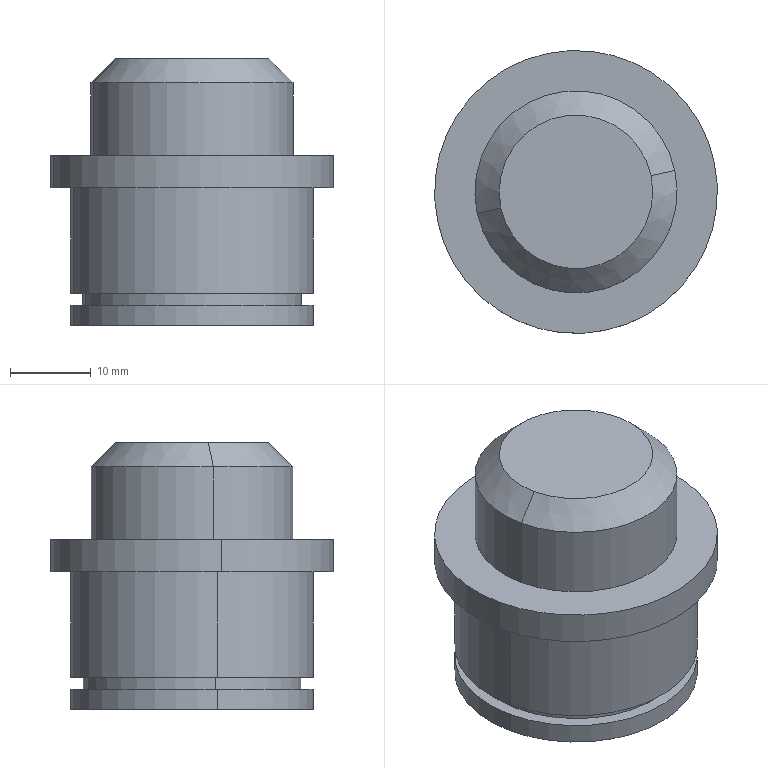Component | SolidWorks | 12AOuterSideWheel-EngravingAndMillingAxis-1_12AOuterSideWheelSmallAxis-1 | 1 solid | 18 faces | box 35 x 35 x 33 mm | volume 21229 mm3 | cylinder 10 | plane 6 | cone 2 | commonest cylinder face diameters 30 x4 27 x2 35 x2 25 x2 | material Cr12MoV
build123d program:
from build123d import *

# Parameters (mm, degrees)
SKETCH1_R           = 12.5
BOSS_EXTRUDE1_DEPTH = 12
SKETCH2_R           = 17.5
BOSS_EXTRUDE2_DEPTH = 4
SKETCH3_R           = 15
BOSS_EXTRUDE3_DEPTH = 17
SKETCH4_W           = 1.5
SKETCH4_H           = 1.5
CHAMFER1_SIZE       = 3


with BuildPart() as part:
    # Sketch1 → Boss-Extrude1 (new body)
    with BuildSketch(Plane.XY):
        Circle(SKETCH1_R)
    extrude(amount=BOSS_EXTRUDE1_DEPTH)

    # Sketch2 → Boss-Extrude2 (add)
    with BuildSketch(Plane.XY.offset(12)):
        Circle(SKETCH2_R)
    extrude(amount=BOSS_EXTRUDE2_DEPTH)

    # Sketch3 → Boss-Extrude3 (add)
    with BuildSketch(Plane.XY.offset(16)):
        Circle(SKETCH3_R)
    extrude(amount=BOSS_EXTRUDE3_DEPTH)

    # Sketch4 → Cut-Revolve1 (revolve, cut)
    with BuildSketch(Plane(origin=(0, 0, 0), x_dir=(1, 0, 0), z_dir=(0, 1, 0))):
        with Locations((14.25, -29.75)):
            Rectangle(SKETCH4_W, SKETCH4_H)
    revolve(axis=Axis((0, 0, 33), (0, 0, -1)), mode=Mode.SUBTRACT)

    # Chamfer1
    chamfer1_edges = [part.edges().sort_by_distance(p)[0] for p in [
        (-12.5, 0, 0),
    ]]
    chamfer(chamfer1_edges, length=CHAMFER1_SIZE)


solid = part.part

# Placed as in the assembly
solid = solid.moved(Location((271.598, 136.538, 72.25), (180, 0, 0)))
STEP:
#1=CARTESIAN_POINT('',(11.058,5.455,2.844));
#2=VERTEX_POINT('',#1);
#3=CARTESIAN_POINT('',(10.327,5.296,2.844));
#4=VERTEX_POINT('',#3);
#5=CARTESIAN_POINT('',(10.693,5.376,2.844));
#6=DIRECTION('',(0.,0.,1.));
#7=DIRECTION('',(-0.9774,-0.2113,0.));
#8=AXIS2_PLACEMENT_3D('',#5,#6,#7);
#9=CIRCLE('',#8,0.374);
#10=EDGE_CURVE('',#2,#4,#9,.T.);
#11=ORIENTED_EDGE('',*,*,#10,.F.);
#12=CARTESIAN_POINT('',(11.174,5.48,2.726));
#13=VERTEX_POINT('',#12);
#14=CARTESIAN_POINT('',(11.174,5.48,2.726));
#15=DIRECTION('',(0.6911,0.1494,-0.7071));
#16=VECTOR('',#15,39.37);
#17=LINE('',#14,#16);
#18=EDGE_CURVE('',#2,#13,#17,.T.);
#19=ORIENTED_EDGE('',*,*,#18,.T.);
#20=CARTESIAN_POINT('',(10.212,5.272,2.726));
#21=VERTEX_POINT('',#20);
#22=CARTESIAN_POINT('',(10.693,5.376,2.726));
#23=DIRECTION('',(0.,0.,-1.));
#24=DIRECTION('',(-0.9774,-0.2113,0.));
#25=AXIS2_PLACEMENT_3D('',#22,#23,#24);
#26=CIRCLE('',#25,0.4921);
#27=EDGE_CURVE('',#21,#13,#26,.T.);
#28=ORIENTED_EDGE('',*,*,#27,.F.);
#29=CARTESIAN_POINT('',(10.212,5.272,2.726));
#30=DIRECTION('',(-0.6911,-0.1494,-0.7071));
#31=VECTOR('',#30,39.37);
#32=LINE('',#29,#31);
#33=EDGE_CURVE('',#4,#21,#32,.T.);
#34=ORIENTED_EDGE('',*,*,#33,.F.);
#35=EDGE_LOOP('',(#11,#19,#28,#34));
#36=FACE_OUTER_BOUND('',#35,.T.);
#37=CARTESIAN_POINT('',(10.693,5.376,2.726));
#38=DIRECTION('',(0.,0.,-1.));
#39=DIRECTION('',(-0.9774,-0.2113,0.));
#40=AXIS2_PLACEMENT_3D('',#37,#38,#39);
#41=CONICAL_SURFACE('',#40,0.4921,0.7854);
#42=ADVANCED_FACE('',(#36),#41,.T.);
#43=CARTESIAN_POINT('',(10.116,5.251,1.545));
#44=VERTEX_POINT('',#43);
#45=CARTESIAN_POINT('',(11.27,5.5,1.545));
#46=VERTEX_POINT('',#45);
#47=CARTESIAN_POINT('',(10.693,5.376,1.545));
#48=DIRECTION('',(0.,0.,-1.));
#49=DIRECTION('',(-0.9774,-0.2113,0.));
#50=AXIS2_PLACEMENT_3D('',#47,#48,#49);
#51=CIRCLE('',#50,0.5906);
#52=EDGE_CURVE('',#44,#46,#51,.T.);
#53=ORIENTED_EDGE('',*,*,#52,.F.);
#54=CARTESIAN_POINT('',(10.116,5.251,1.644));
#55=VERTEX_POINT('',#54);
#56=CARTESIAN_POINT('',(10.116,5.251,1.545));
#57=DIRECTION('',(0.,0.,1.));
#58=VECTOR('',#57,39.37);
#59=LINE('',#56,#58);
#60=EDGE_CURVE('',#44,#55,#59,.T.);
#61=ORIENTED_EDGE('',*,*,#60,.T.);
#62=CARTESIAN_POINT('',(11.27,5.5,1.644));
#63=VERTEX_POINT('',#62);
#64=CARTESIAN_POINT('',(10.693,5.376,1.644));
#65=DIRECTION('',(0.,0.,-1.));
#66=DIRECTION('',(-0.9774,-0.2113,0.));
#67=AXIS2_PLACEMENT_3D('',#64,#65,#66);
#68=CIRCLE('',#67,0.5906);
#69=EDGE_CURVE('',#55,#63,#68,.T.);
#70=ORIENTED_EDGE('',*,*,#69,.T.);
#71=CARTESIAN_POINT('',(11.27,5.5,1.545));
#72=DIRECTION('',(0.,0.,1.));
#73=VECTOR('',#72,39.37);
#74=LINE('',#71,#73);
#75=EDGE_CURVE('',#46,#63,#74,.T.);
#76=ORIENTED_EDGE('',*,*,#75,.F.);
#77=EDGE_LOOP('',(#53,#61,#70,#76));
#78=FACE_OUTER_BOUND('',#77,.T.);
#79=CARTESIAN_POINT('',(10.693,5.376,1.545));
#80=DIRECTION('',(0.,0.,1.));
#81=DIRECTION('',(0.9774,0.2113,0.));
#82=AXIS2_PLACEMENT_3D('',#79,#80,#81);
#83=CYLINDRICAL_SURFACE('',#82,0.5906);
#84=ADVANCED_FACE('',(#78),#83,.T.);
#85=CARTESIAN_POINT('',(10.173,5.263,1.703));
#86=VERTEX_POINT('',#85);
#87=CARTESIAN_POINT('',(11.212,5.488,1.703));
#88=VERTEX_POINT('',#87);
#89=CARTESIAN_POINT('',(10.693,5.376,1.703));
#90=DIRECTION('',(0.,0.,-1.));
#91=DIRECTION('',(-0.9774,-0.2113,0.));
#92=AXIS2_PLACEMENT_3D('',#89,#90,#91);
#93=CIRCLE('',#92,0.5315);
#94=EDGE_CURVE('',#86,#88,#93,.T.);
#95=ORIENTED_EDGE('',*,*,#94,.T.);
#96=CARTESIAN_POINT('',(11.212,5.488,1.644));
#97=VERTEX_POINT('',#96);
#98=CARTESIAN_POINT('',(11.212,5.488,1.545));
#99=DIRECTION('',(0.,0.,-1.));
#100=VECTOR('',#99,39.37);
#101=LINE('',#98,#100);
#102=EDGE_CURVE('',#88,#97,#101,.T.);
#103=ORIENTED_EDGE('',*,*,#102,.T.);
#104=CARTESIAN_POINT('',(10.173,5.263,1.644));
#105=VERTEX_POINT('',#104);
#106=CARTESIAN_POINT('',(10.693,5.376,1.644));
#107=DIRECTION('',(0.,0.,-1.));
#108=DIRECTION('',(-0.9774,-0.2113,0.));
#109=AXIS2_PLACEMENT_3D('',#106,#107,#108);
#110=CIRCLE('',#109,0.5315);
#111=EDGE_CURVE('',#105,#97,#110,.T.);
#112=ORIENTED_EDGE('',*,*,#111,.F.);
#113=CARTESIAN_POINT('',(10.173,5.263,1.545));
#114=DIRECTION('',(0.,0.,-1.));
#115=VECTOR('',#114,39.37);
#116=LINE('',#113,#115);
#117=EDGE_CURVE('',#86,#105,#116,.T.);
#118=ORIENTED_EDGE('',*,*,#117,.F.);
#119=EDGE_LOOP('',(#95,#103,#112,#118));
#120=FACE_OUTER_BOUND('',#119,.T.);
#121=CARTESIAN_POINT('',(10.693,5.376,1.545));
#122=DIRECTION('',(0.,0.,-1.));
#123=DIRECTION('',(-0.9774,-0.2113,0.));
#124=AXIS2_PLACEMENT_3D('',#121,#122,#123);
#125=CYLINDRICAL_SURFACE('',#124,0.5315);
#126=ADVANCED_FACE('',(#120),#125,.T.);
#127=CARTESIAN_POINT('',(10.019,5.23,2.215));
#128=VERTEX_POINT('',#127);
#129=CARTESIAN_POINT('',(11.366,5.521,2.215));
#130=VERTEX_POINT('',#129);
#131=CARTESIAN_POINT('',(10.693,5.376,2.215));
#132=DIRECTION('',(0.,0.,-1.));
#133=DIRECTION('',(-0.9774,-0.2113,0.));
#134=AXIS2_PLACEMENT_3D('',#131,#132,#133);
#135=CIRCLE('',#134,0.689);
#136=EDGE_CURVE('',#128,#130,#135,.T.);
#137=ORIENTED_EDGE('',*,*,#136,.F.);
#138=CARTESIAN_POINT('',(10.019,5.23,2.372));
#139=VERTEX_POINT('',#138);
#140=CARTESIAN_POINT('',(10.019,5.23,2.215));
#141=DIRECTION('',(0.,0.,1.));
#142=VECTOR('',#141,39.37);
#143=LINE('',#140,#142);
#144=EDGE_CURVE('',#128,#139,#143,.T.);
#145=ORIENTED_EDGE('',*,*,#144,.T.);
#146=CARTESIAN_POINT('',(11.366,5.521,2.372));
#147=VERTEX_POINT('',#146);
#148=CARTESIAN_POINT('',(10.693,5.376,2.372));
#149=DIRECTION('',(0.,0.,-1.));
#150=DIRECTION('',(-0.9774,-0.2113,0.));
#151=AXIS2_PLACEMENT_3D('',#148,#149,#150);
#152=CIRCLE('',#151,0.689);
#153=EDGE_CURVE('',#139,#147,#152,.T.);
#154=ORIENTED_EDGE('',*,*,#153,.T.);
#155=CARTESIAN_POINT('',(11.366,5.521,2.215));
#156=DIRECTION('',(0.,0.,1.));
#157=VECTOR('',#156,39.37);
#158=LINE('',#155,#157);
#159=EDGE_CURVE('',#130,#147,#158,.T.);
#160=ORIENTED_EDGE('',*,*,#159,.F.);
#161=EDGE_LOOP('',(#137,#145,#154,#160));
#162=FACE_OUTER_BOUND('',#161,.T.);
#163=CARTESIAN_POINT('',(10.693,5.376,2.215));
#164=DIRECTION('',(0.,0.,1.));
#165=DIRECTION('',(0.9774,0.2113,0.));
#166=AXIS2_PLACEMENT_3D('',#163,#164,#165);
#167=CYLINDRICAL_SURFACE('',#166,0.689);
#168=ADVANCED_FACE('',(#162),#167,.T.);
#169=CARTESIAN_POINT('',(10.212,5.272,2.372));
#170=VERTEX_POINT('',#169);
#171=CARTESIAN_POINT('',(11.174,5.48,2.372));
#172=VERTEX_POINT('',#171);
#173=CARTESIAN_POINT('',(10.693,5.376,2.372));
#174=DIRECTION('',(0.,0.,-1.));
#175=DIRECTION('',(-0.9774,-0.2113,0.));
#176=AXIS2_PLACEMENT_3D('',#173,#174,#175);
#177=CIRCLE('',#176,0.4921);
#178=EDGE_CURVE('',#170,#172,#177,.T.);
#179=ORIENTED_EDGE('',*,*,#178,.F.);
#180=CARTESIAN_POINT('',(10.212,5.272,2.372));
#181=DIRECTION('',(0.,0.,1.));
#182=VECTOR('',#181,39.37);
#183=LINE('',#180,#182);
#184=EDGE_CURVE('',#170,#21,#183,.T.);
#185=ORIENTED_EDGE('',*,*,#184,.T.);
#186=ORIENTED_EDGE('',*,*,#27,.T.);
#187=CARTESIAN_POINT('',(11.174,5.48,2.372));
#188=DIRECTION('',(0.,0.,1.));
#189=VECTOR('',#188,39.37);
#190=LINE('',#187,#189);
#191=EDGE_CURVE('',#172,#13,#190,.T.);
#192=ORIENTED_EDGE('',*,*,#191,.F.);
#193=EDGE_LOOP('',(#179,#185,#186,#192));
#194=FACE_OUTER_BOUND('',#193,.T.);
#195=CARTESIAN_POINT('',(10.693,5.376,2.372));
#196=DIRECTION('',(0.,0.,1.));
#197=DIRECTION('',(0.9774,0.2113,0.));
#198=AXIS2_PLACEMENT_3D('',#195,#196,#197);
#199=CYLINDRICAL_SURFACE('',#198,0.4921);
#200=ADVANCED_FACE('',(#194),#199,.T.);
#201=CARTESIAN_POINT('',(10.116,5.251,1.703));
#202=VERTEX_POINT('',#201);
#203=CARTESIAN_POINT('',(11.27,5.5,1.703));
#204=VERTEX_POINT('',#203);
#205=CARTESIAN_POINT('',(10.693,5.376,1.703));
#206=DIRECTION('',(0.,0.,-1.));
#207=DIRECTION('',(-0.9774,-0.2113,0.));
#208=AXIS2_PLACEMENT_3D('',#205,#206,#207);
#209=CIRCLE('',#208,0.5906);
#210=EDGE_CURVE('',#202,#204,#209,.T.);
#211=ORIENTED_EDGE('',*,*,#210,.F.);
#212=CARTESIAN_POINT('',(10.116,5.251,2.215));
#213=VERTEX_POINT('',#212);
#214=CARTESIAN_POINT('',(10.116,5.251,1.545));
#215=DIRECTION('',(0.,0.,1.));
#216=VECTOR('',#215,39.37);
#217=LINE('',#214,#216);
#218=EDGE_CURVE('',#202,#213,#217,.T.);
#219=ORIENTED_EDGE('',*,*,#218,.T.);
#220=CARTESIAN_POINT('',(11.27,5.5,2.215));
#221=VERTEX_POINT('',#220);
#222=CARTESIAN_POINT('',(10.693,5.376,2.215));
#223=DIRECTION('',(0.,0.,-1.));
#224=DIRECTION('',(-0.9774,-0.2113,0.));
#225=AXIS2_PLACEMENT_3D('',#222,#223,#224);
#226=CIRCLE('',#225,0.5906);
#227=EDGE_CURVE('',#213,#221,#226,.T.);
#228=ORIENTED_EDGE('',*,*,#227,.T.);
#229=CARTESIAN_POINT('',(11.27,5.5,1.545));
#230=DIRECTION('',(0.,0.,1.));
#231=VECTOR('',#230,39.37);
#232=LINE('',#229,#231);
#233=EDGE_CURVE('',#204,#221,#232,.T.);
#234=ORIENTED_EDGE('',*,*,#233,.F.);
#235=EDGE_LOOP('',(#211,#219,#228,#234));
#236=FACE_OUTER_BOUND('',#235,.T.);
#237=CARTESIAN_POINT('',(10.693,5.376,1.545));
#238=DIRECTION('',(0.,0.,1.));
#239=DIRECTION('',(0.9774,0.2113,0.));
#240=AXIS2_PLACEMENT_3D('',#237,#238,#239);
#241=CYLINDRICAL_SURFACE('',#240,0.5906);
#242=ADVANCED_FACE('',(#236),#241,.T.);
#243=ORIENTED_EDGE('',*,*,#218,.F.);
#244=CARTESIAN_POINT('',(10.693,5.376,1.703));
#245=DIRECTION('',(0.,0.,-1.));
#246=DIRECTION('',(-0.9774,-0.2113,0.));
#247=AXIS2_PLACEMENT_3D('',#244,#245,#246);
#248=CIRCLE('',#247,0.5906);
#249=EDGE_CURVE('',#204,#202,#248,.T.);
#250=ORIENTED_EDGE('',*,*,#249,.F.);
#251=ORIENTED_EDGE('',*,*,#233,.T.);
#252=CARTESIAN_POINT('',(10.693,5.376,2.215));
#253=DIRECTION('',(0.,0.,-1.));
#254=DIRECTION('',(-0.9774,-0.2113,0.));
#255=AXIS2_PLACEMENT_3D('',#252,#253,#254);
#256=CIRCLE('',#255,0.5906);
#257=EDGE_CURVE('',#221,#213,#256,.T.);
#258=ORIENTED_EDGE('',*,*,#257,.T.);
#259=EDGE_LOOP('',(#243,#250,#251,#258));
#260=FACE_OUTER_BOUND('',#259,.T.);
#261=CARTESIAN_POINT('',(10.693,5.376,1.545));
#262=DIRECTION('',(0.,0.,1.));
#263=DIRECTION('',(0.9774,0.2113,0.));
#264=AXIS2_PLACEMENT_3D('',#261,#262,#263);
#265=CYLINDRICAL_SURFACE('',#264,0.5906);
#266=ADVANCED_FACE('',(#260),#265,.T.);
#267=ORIENTED_EDGE('',*,*,#184,.F.);
#268=CARTESIAN_POINT('',(10.693,5.376,2.372));
#269=DIRECTION('',(0.,0.,-1.));
#270=DIRECTION('',(-0.9774,-0.2113,0.));
#271=AXIS2_PLACEMENT_3D('',#268,#269,#270);
#272=CIRCLE('',#271,0.4921);
#273=EDGE_CURVE('',#172,#170,#272,.T.);
#274=ORIENTED_EDGE('',*,*,#273,.F.);
#275=ORIENTED_EDGE('',*,*,#191,.T.);
#276=CARTESIAN_POINT('',(10.693,5.376,2.726));
#277=DIRECTION('',(0.,0.,-1.));
#278=DIRECTION('',(-0.9774,-0.2113,0.));
#279=AXIS2_PLACEMENT_3D('',#276,#277,#278);
#280=CIRCLE('',#279,0.4921);
#281=EDGE_CURVE('',#13,#21,#280,.T.);
#282=ORIENTED_EDGE('',*,*,#281,.T.);
#283=EDGE_LOOP('',(#267,#274,#275,#282));
#284=FACE_OUTER_BOUND('',#283,.T.);
#285=CARTESIAN_POINT('',(10.693,5.376,2.372));
#286=DIRECTION('',(0.,0.,1.));
#287=DIRECTION('',(0.9774,0.2113,0.));
#288=AXIS2_PLACEMENT_3D('',#285,#286,#287);
#289=CYLINDRICAL_SURFACE('',#288,0.4921);
#290=ADVANCED_FACE('',(#284),#289,.T.);
#291=CARTESIAN_POINT('',(10.693,5.376,2.844));
#292=DIRECTION('',(0.,0.,1.));
#293=DIRECTION('',(-0.9774,-0.2113,0.));
#294=AXIS2_PLACEMENT_3D('',#291,#292,#293);
#295=CIRCLE('',#294,0.374);
#296=EDGE_CURVE('',#4,#2,#295,.T.);
#297=ORIENTED_EDGE('',*,*,#296,.T.);
#298=ORIENTED_EDGE('',*,*,#10,.T.);
#299=EDGE_LOOP('',(#297,#298));
#300=FACE_OUTER_BOUND('',#299,.T.);
#301=CARTESIAN_POINT('',(10.693,5.376,2.844));
#302=DIRECTION('',(0.,0.,-1.));
#303=DIRECTION('',(-0.9774,-0.2113,0.));
#304=AXIS2_PLACEMENT_3D('',#301,#302,#303);
#305=PLANE('',#304);
#306=ADVANCED_FACE('',(#300),#305,.F.);
#307=ORIENTED_EDGE('',*,*,#144,.F.);
#308=CARTESIAN_POINT('',(10.693,5.376,2.215));
#309=DIRECTION('',(0.,0.,-1.));
#310=DIRECTION('',(-0.9774,-0.2113,0.));
#311=AXIS2_PLACEMENT_3D('',#308,#309,#310);
#312=CIRCLE('',#311,0.689);
#313=EDGE_CURVE('',#130,#128,#312,.T.);
#314=ORIENTED_EDGE('',*,*,#313,.F.);
#315=ORIENTED_EDGE('',*,*,#159,.T.);
#316=CARTESIAN_POINT('',(10.693,5.376,2.372));
#317=DIRECTION('',(0.,0.,-1.));
#318=DIRECTION('',(-0.9774,-0.2113,0.));
#319=AXIS2_PLACEMENT_3D('',#316,#317,#318);
#320=CIRCLE('',#319,0.689);
#321=EDGE_CURVE('',#147,#139,#320,.T.);
#322=ORIENTED_EDGE('',*,*,#321,.T.);
#323=EDGE_LOOP('',(#307,#314,#315,#322));
#324=FACE_OUTER_BOUND('',#323,.T.);
#325=CARTESIAN_POINT('',(10.693,5.376,2.215));
#326=DIRECTION('',(0.,0.,1.));
#327=DIRECTION('',(0.9774,0.2113,0.));
#328=AXIS2_PLACEMENT_3D('',#325,#326,#327);
#329=CYLINDRICAL_SURFACE('',#328,0.689);
#330=ADVANCED_FACE('',(#324),#329,.T.);
#331=ORIENTED_EDGE('',*,*,#257,.F.);
#332=ORIENTED_EDGE('',*,*,#227,.F.);
#333=EDGE_LOOP('',(#331,#332));
#334=FACE_BOUND('',#333,.T.);
#335=ORIENTED_EDGE('',*,*,#313,.T.);
#336=ORIENTED_EDGE('',*,*,#136,.T.);
#337=EDGE_LOOP('',(#335,#336));
#338=FACE_OUTER_BOUND('',#337,.T.);
#339=CARTESIAN_POINT('',(10.693,5.376,2.215));
#340=DIRECTION('',(0.,0.,-1.));
#341=DIRECTION('',(-0.9774,-0.2113,0.));
#342=AXIS2_PLACEMENT_3D('',#339,#340,#341);
#343=PLANE('',#342);
#344=ADVANCED_FACE('',(#334,#338),#343,.T.);
#345=ORIENTED_EDGE('',*,*,#273,.T.);
#346=ORIENTED_EDGE('',*,*,#178,.T.);
#347=EDGE_LOOP('',(#345,#346));
#348=FACE_BOUND('',#347,.T.);
#349=ORIENTED_EDGE('',*,*,#321,.F.);
#350=ORIENTED_EDGE('',*,*,#153,.F.);
#351=EDGE_LOOP('',(#349,#350));
#352=FACE_OUTER_BOUND('',#351,.T.);
#353=CARTESIAN_POINT('',(10.693,5.376,2.372));
#354=DIRECTION('',(0.,0.,-1.));
#355=DIRECTION('',(-0.9774,-0.2113,0.));
#356=AXIS2_PLACEMENT_3D('',#353,#354,#355);
#357=PLANE('',#356);
#358=ADVANCED_FACE('',(#348,#352),#357,.F.);
#359=ORIENTED_EDGE('',*,*,#94,.F.);
#360=CARTESIAN_POINT('',(10.693,5.376,1.703));
#361=DIRECTION('',(0.,0.,-1.));
#362=DIRECTION('',(-0.9774,-0.2113,0.));
#363=AXIS2_PLACEMENT_3D('',#360,#361,#362);
#364=CIRCLE('',#363,0.5315);
#365=EDGE_CURVE('',#88,#86,#364,.T.);
#366=ORIENTED_EDGE('',*,*,#365,.F.);
#367=EDGE_LOOP('',(#359,#366));
#368=FACE_BOUND('',#367,.T.);
#369=ORIENTED_EDGE('',*,*,#249,.T.);
#370=ORIENTED_EDGE('',*,*,#210,.T.);
#371=EDGE_LOOP('',(#369,#370));
#372=FACE_OUTER_BOUND('',#371,.T.);
#373=CARTESIAN_POINT('',(10.116,5.251,1.703));
#374=DIRECTION('',(0.,0.,1.));
#375=DIRECTION('',(0.9774,0.2113,0.));
#376=AXIS2_PLACEMENT_3D('',#373,#374,#375);
#377=PLANE('',#376);
#378=ADVANCED_FACE('',(#368,#372),#377,.F.);
#379=ORIENTED_EDGE('',*,*,#102,.F.);
#380=ORIENTED_EDGE('',*,*,#365,.T.);
#381=ORIENTED_EDGE('',*,*,#117,.T.);
#382=CARTESIAN_POINT('',(10.693,5.376,1.644));
#383=DIRECTION('',(0.,0.,-1.));
#384=DIRECTION('',(-0.9774,-0.2113,0.));
#385=AXIS2_PLACEMENT_3D('',#382,#383,#384);
#386=CIRCLE('',#385,0.5315);
#387=EDGE_CURVE('',#97,#105,#386,.T.);
#388=ORIENTED_EDGE('',*,*,#387,.F.);
#389=EDGE_LOOP('',(#379,#380,#381,#388));
#390=FACE_OUTER_BOUND('',#389,.T.);
#391=CARTESIAN_POINT('',(10.693,5.376,1.545));
#392=DIRECTION('',(0.,0.,-1.));
#393=DIRECTION('',(-0.9774,-0.2113,0.));
#394=AXIS2_PLACEMENT_3D('',#391,#392,#393);
#395=CYLINDRICAL_SURFACE('',#394,0.5315);
#396=ADVANCED_FACE('',(#390),#395,.T.);
#397=CARTESIAN_POINT('',(10.693,5.376,1.644));
#398=DIRECTION('',(0.,0.,-1.));
#399=DIRECTION('',(-0.9774,-0.2113,0.));
#400=AXIS2_PLACEMENT_3D('',#397,#398,#399);
#401=CIRCLE('',#400,0.5906);
#402=EDGE_CURVE('',#63,#55,#401,.T.);
#403=ORIENTED_EDGE('',*,*,#402,.F.);
#404=ORIENTED_EDGE('',*,*,#69,.F.);
#405=EDGE_LOOP('',(#403,#404));
#406=FACE_OUTER_BOUND('',#405,.T.);
#407=ORIENTED_EDGE('',*,*,#111,.T.);
#408=ORIENTED_EDGE('',*,*,#387,.T.);
#409=EDGE_LOOP('',(#407,#408));
#410=FACE_BOUND('',#409,.T.);
#411=CARTESIAN_POINT('',(10.116,5.251,1.644));
#412=DIRECTION('',(0.,0.,-1.));
#413=DIRECTION('',(-0.9774,-0.2113,0.));
#414=AXIS2_PLACEMENT_3D('',#411,#412,#413);
#415=PLANE('',#414);
#416=ADVANCED_FACE('',(#406,#410),#415,.F.);
#417=CARTESIAN_POINT('',(10.693,5.376,1.545));
#418=DIRECTION('',(0.,0.,-1.));
#419=DIRECTION('',(-0.9774,-0.2113,0.));
#420=AXIS2_PLACEMENT_3D('',#417,#418,#419);
#421=CIRCLE('',#420,0.5906);
#422=EDGE_CURVE('',#46,#44,#421,.T.);
#423=ORIENTED_EDGE('',*,*,#422,.T.);
#424=ORIENTED_EDGE('',*,*,#52,.T.);
#425=EDGE_LOOP('',(#423,#424));
#426=FACE_OUTER_BOUND('',#425,.T.);
#427=CARTESIAN_POINT('',(10.693,5.376,1.545));
#428=DIRECTION('',(0.,0.,-1.));
#429=DIRECTION('',(-0.9774,-0.2113,0.));
#430=AXIS2_PLACEMENT_3D('',#427,#428,#429);
#431=PLANE('',#430);
#432=ADVANCED_FACE('',(#426),#431,.T.);
#433=ORIENTED_EDGE('',*,*,#60,.F.);
#434=ORIENTED_EDGE('',*,*,#422,.F.);
#435=ORIENTED_EDGE('',*,*,#75,.T.);
#436=ORIENTED_EDGE('',*,*,#402,.T.);
#437=EDGE_LOOP('',(#433,#434,#435,#436));
#438=FACE_OUTER_BOUND('',#437,.T.);
#439=CARTESIAN_POINT('',(10.693,5.376,1.545));
#440=DIRECTION('',(0.,0.,1.));
#441=DIRECTION('',(0.9774,0.2113,0.));
#442=AXIS2_PLACEMENT_3D('',#439,#440,#441);
#443=CYLINDRICAL_SURFACE('',#442,0.5906);
#444=ADVANCED_FACE('',(#438),#443,.T.);
#445=ORIENTED_EDGE('',*,*,#18,.F.);
#446=ORIENTED_EDGE('',*,*,#296,.F.);
#447=ORIENTED_EDGE('',*,*,#33,.T.);
#448=ORIENTED_EDGE('',*,*,#281,.F.);
#449=EDGE_LOOP('',(#445,#446,#447,#448));
#450=FACE_OUTER_BOUND('',#449,.T.);
#451=CARTESIAN_POINT('',(10.693,5.376,2.726));
#452=DIRECTION('',(0.,0.,-1.));
#453=DIRECTION('',(-0.9774,-0.2113,0.));
#454=AXIS2_PLACEMENT_3D('',#451,#452,#453);
#455=CONICAL_SURFACE('',#454,0.4921,0.7854);
#456=ADVANCED_FACE('',(#450),#455,.T.);
#457=CLOSED_SHELL('',(#42,#84,#126,#168,#200,#242,#266,#290,#306,#330,#344,#358,#378,#396,#416,#432,#444,#456));
#458=MANIFOLD_SOLID_BREP('',#457);
#459=CARTESIAN_POINT('',(0.,0.,0.));
#460=DIRECTION('',(0.,0.,1.));
#461=DIRECTION('',(1.,0.,0.));
#462=AXIS2_PLACEMENT_3D('',#459,#460,#461);
#463=(LENGTH_UNIT()NAMED_UNIT(*)SI_UNIT($,.METRE.));
#464=LENGTH_MEASURE_WITH_UNIT(LENGTH_MEASURE(0.0254),#463);
#465=DIMENSIONAL_EXPONENTS(1.,0.,0.,0.,0.,0.,0.);
#466=(CONVERSION_BASED_UNIT('',#464)LENGTH_UNIT()NAMED_UNIT(#465));
#467=UNCERTAINTY_MEASURE_WITH_UNIT(LENGTH_MEASURE(0.00001),#466,'','');
#468=(NAMED_UNIT(*)PLANE_ANGLE_UNIT()SI_UNIT($,.RADIAN.));
#469=(NAMED_UNIT(*)SI_UNIT($,.STERADIAN.)SOLID_ANGLE_UNIT());
#470=(GEOMETRIC_REPRESENTATION_CONTEXT(3)GLOBAL_UNCERTAINTY_ASSIGNED_CONTEXT((#467))GLOBAL_UNIT_ASSIGNED_CONTEXT((#466,#468,#469))REPRESENTATION_CONTEXT('',''));
#471=ADVANCED_BREP_SHAPE_REPRESENTATION('',(#458,#462),#470);
#472=COLOUR_RGB('',0.7922,0.8196,0.9333);
#473=FILL_AREA_STYLE_COLOUR('',#472);
#474=FILL_AREA_STYLE('',(#473));
#475=SURFACE_STYLE_FILL_AREA(#474);
#476=SURFACE_SIDE_STYLE('',(#475));
#477=SURFACE_STYLE_USAGE(.BOTH.,#476);
#478=PRESENTATION_STYLE_ASSIGNMENT((#477));
#479=STYLED_ITEM('',(#478),#458);
#480=PRESENTATION_LAYER_ASSIGNMENT('','',(#479));
#481=(LENGTH_UNIT()NAMED_UNIT(*)SI_UNIT($,.METRE.));
#482=LENGTH_MEASURE_WITH_UNIT(LENGTH_MEASURE(0.0254),#481);
#483=DIMENSIONAL_EXPONENTS(1.,0.,0.,0.,0.,0.,0.);
#484=(CONVERSION_BASED_UNIT('',#482)LENGTH_UNIT()NAMED_UNIT(#483));
#485=UNCERTAINTY_MEASURE_WITH_UNIT(LENGTH_MEASURE(0.00001),#484,'','');
#486=(NAMED_UNIT(*)PLANE_ANGLE_UNIT()SI_UNIT($,.RADIAN.));
#487=(NAMED_UNIT(*)SI_UNIT($,.STERADIAN.)SOLID_ANGLE_UNIT());
#488=(GEOMETRIC_REPRESENTATION_CONTEXT(3)GLOBAL_UNCERTAINTY_ASSIGNED_CONTEXT((#485))GLOBAL_UNIT_ASSIGNED_CONTEXT((#484,#486,#487))REPRESENTATION_CONTEXT('',''));
#489=MECHANICAL_DESIGN_GEOMETRIC_PRESENTATION_REPRESENTATION('',(#479),#488);